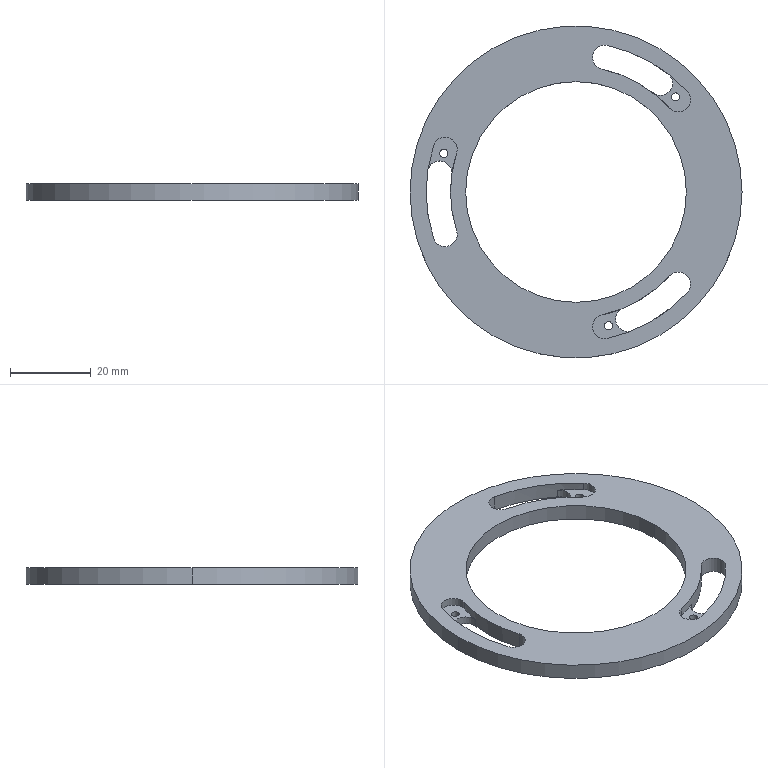CAM job | Mastercam | mm | 9 operations | part box 82 x 82 x 4
1. 2D High Speed (2D Dynamic Mill) | 12 - 12 平铣刀
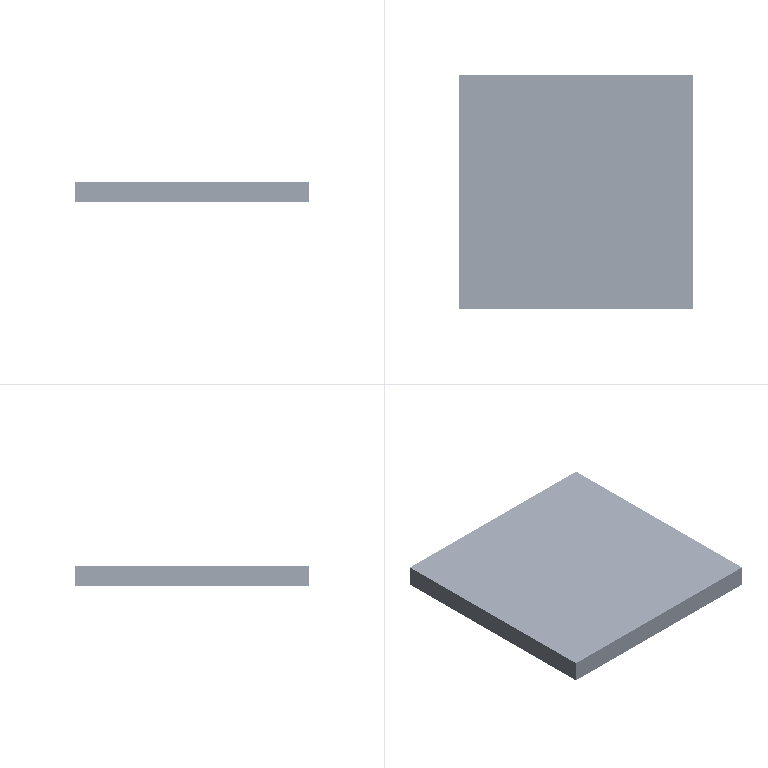2. 2D High Speed (2D Area Mill) | 12 - 12 平铣刀
3. 3D High Speed (Area roughing) | 4 - 4 平铣刀
4. Contour (Ramp) | 5 - 4 平铣刀
5. Contour (2D) | 5 - 4 平铣刀
6. Contour (2D) | 8 - 8 平铣刀
7. Contour (2D) | 8 - 8 平铣刀
8. Contour (2D chamfer) | 7 - 4 倒角刀
9. Drill/Counterbore | 7 - 4 倒角刀